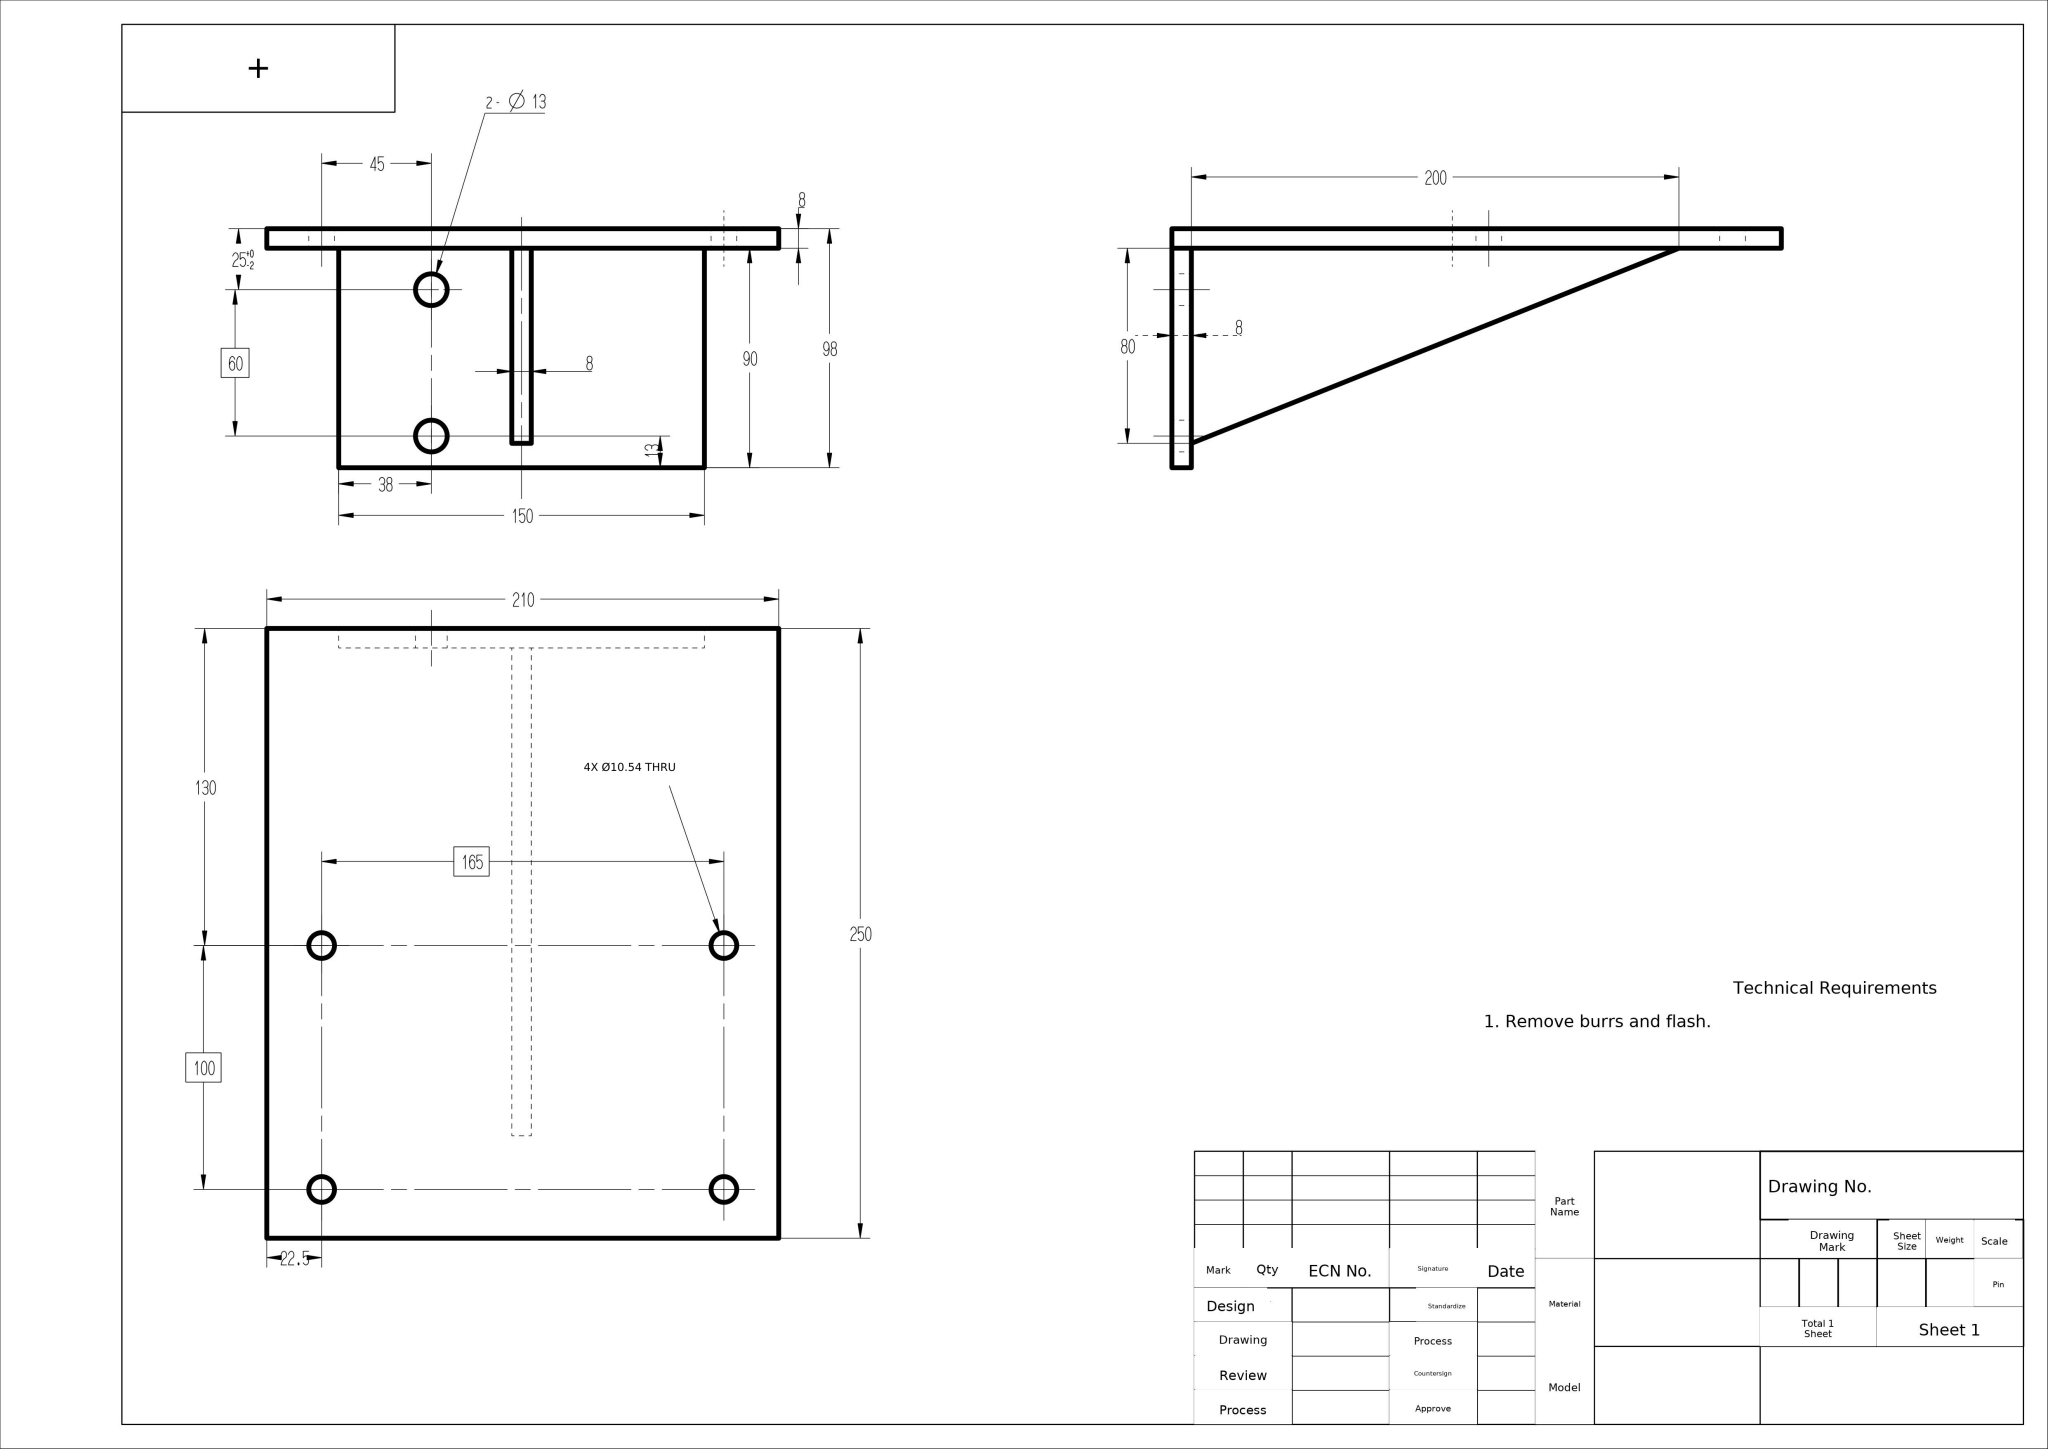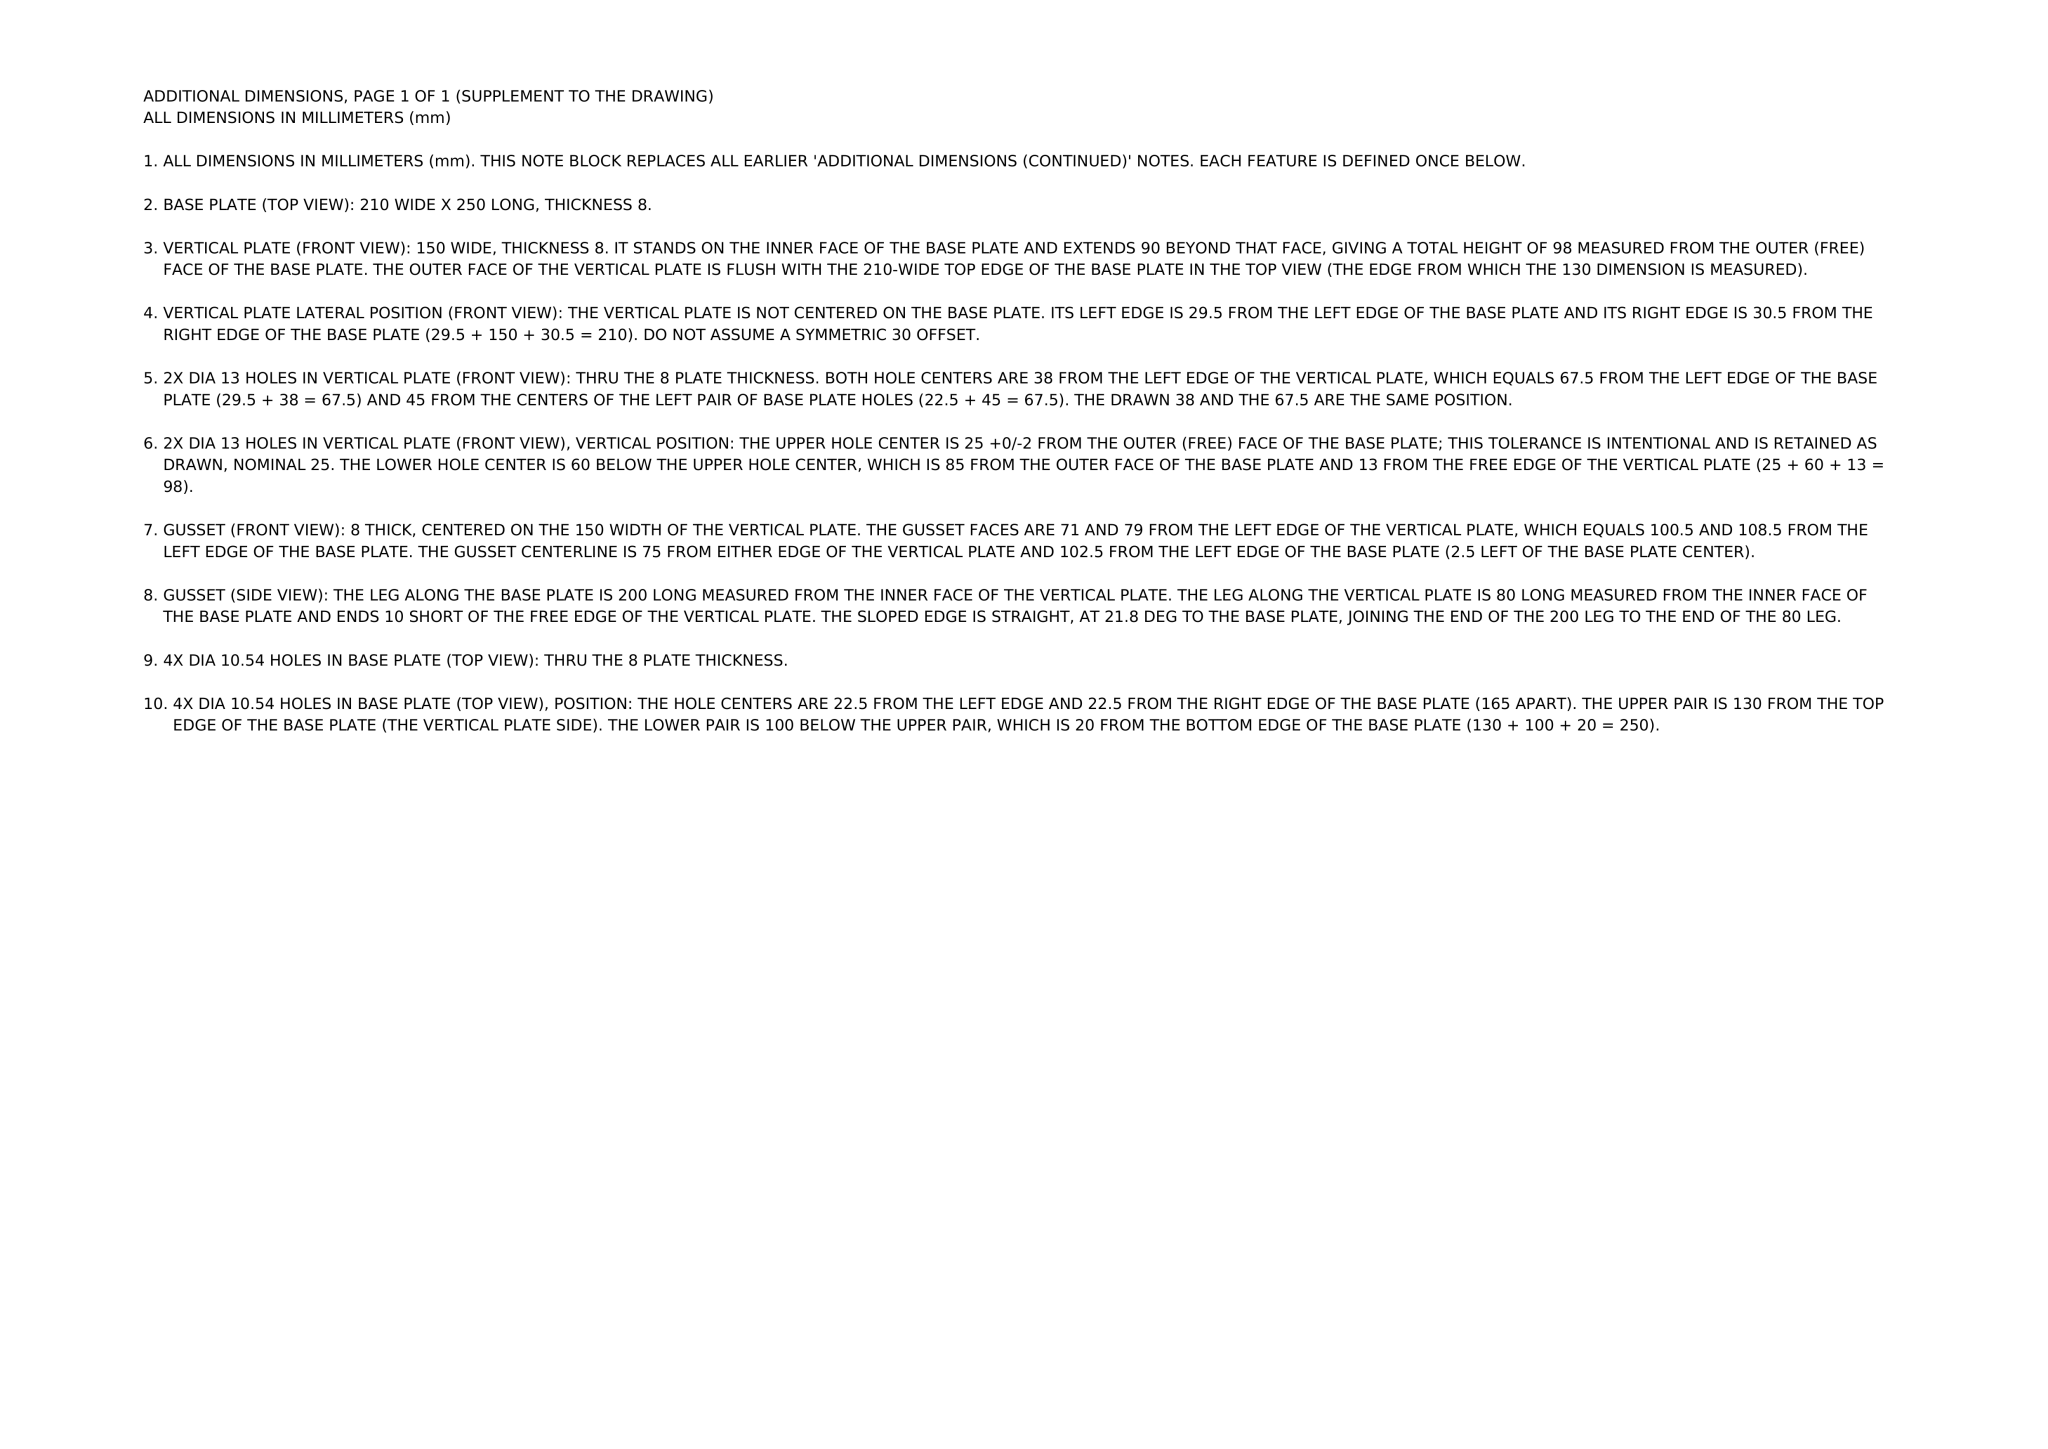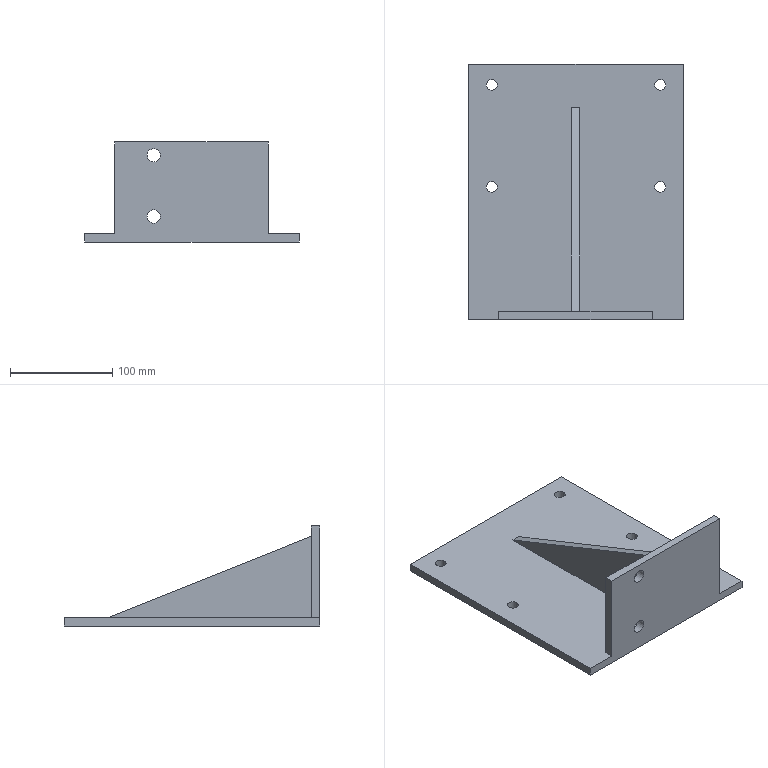Part | NX | mm | 1 solid | 19 faces | box 210 x 250 x 98 mm | volume 587086 mm3 | plane 13 | cylinder 6 | commonest cylinder face diameters 10.536 x4 13 x2
STEP:
#1=CARTESIAN_POINT('',(0.,0.,0.));
#2=DIRECTION('',(0.,0.,1.));
#3=DIRECTION('',(1.,0.,0.));
#4=AXIS2_PLACEMENT_3D('',#1,#2,#3);
#5=(LENGTH_UNIT()NAMED_UNIT(*)SI_UNIT(.MILLI.,.METRE.));
#6=UNCERTAINTY_MEASURE_WITH_UNIT(LENGTH_MEASURE(0.00002),#5,'','');
#7=(NAMED_UNIT(*)PLANE_ANGLE_UNIT()SI_UNIT($,.RADIAN.));
#8=PLANE_ANGLE_MEASURE_WITH_UNIT(PLANE_ANGLE_MEASURE(0.01745),#7);
#9=DIMENSIONAL_EXPONENTS(0.,0.,0.,0.,0.,0.,0.);
#10=(CONVERSION_BASED_UNIT('',#8)NAMED_UNIT(#9)PLANE_ANGLE_UNIT());
#11=(NAMED_UNIT(*)SI_UNIT($,.STERADIAN.)SOLID_ANGLE_UNIT());
#12=(GEOMETRIC_REPRESENTATION_CONTEXT(3)GLOBAL_UNCERTAINTY_ASSIGNED_CONTEXT((#6))GLOBAL_UNIT_ASSIGNED_CONTEXT((#5,#10,#11))REPRESENTATION_CONTEXT('',''));
#13=SHAPE_REPRESENTATION('',(#4),#12);
#14=CARTESIAN_POINT('',(72.,-239.1,85.));
#15=VERTEX_POINT('',#14);
#16=CARTESIAN_POINT('',(65.5,-239.1,85.));
#17=DIRECTION('',(0.,-1.,0.));
#18=DIRECTION('',(1.,0.,0.));
#19=AXIS2_PLACEMENT_3D('',#16,#17,#18);
#20=CIRCLE('',#19,6.5);
#21=EDGE_CURVE('',#15,#15,#20,.T.);
#22=ORIENTED_EDGE('',*,*,#21,.T.);
#23=EDGE_LOOP('',(#22));
#24=FACE_BOUND('',#23,.T.);
#25=CARTESIAN_POINT('',(72.,-239.1,25.));
#26=VERTEX_POINT('',#25);
#27=CARTESIAN_POINT('',(65.5,-239.1,25.));
#28=DIRECTION('',(0.,-1.,0.));
#29=DIRECTION('',(1.,0.,0.));
#30=AXIS2_PLACEMENT_3D('',#27,#28,#29);
#31=CIRCLE('',#30,6.5);
#32=EDGE_CURVE('',#26,#26,#31,.T.);
#33=ORIENTED_EDGE('',*,*,#32,.T.);
#34=EDGE_LOOP('',(#33));
#35=FACE_BOUND('',#34,.T.);
#36=CARTESIAN_POINT('',(177.5,-239.1,8.));
#37=VERTEX_POINT('',#36);
#38=CARTESIAN_POINT('',(106.5,-239.1,8.));
#39=VERTEX_POINT('',#38);
#40=CARTESIAN_POINT('',(177.5,-239.1,8.));
#41=DIRECTION('',(-1.,0.,0.));
#42=VECTOR('',#41,1.);
#43=LINE('',#40,#42);
#44=EDGE_CURVE('',#37,#39,#43,.T.);
#45=ORIENTED_EDGE('',*,*,#44,.T.);
#46=CARTESIAN_POINT('',(106.5,-239.1,88.));
#47=VERTEX_POINT('',#46);
#48=CARTESIAN_POINT('',(106.5,-239.1,8.));
#49=DIRECTION('',(0.,0.,1.));
#50=VECTOR('',#49,1.);
#51=LINE('',#48,#50);
#52=EDGE_CURVE('',#39,#47,#51,.T.);
#53=ORIENTED_EDGE('',*,*,#52,.T.);
#54=CARTESIAN_POINT('',(98.5,-239.1,88.));
#55=VERTEX_POINT('',#54);
#56=CARTESIAN_POINT('',(106.5,-239.1,88.));
#57=DIRECTION('',(-1.,0.,0.));
#58=VECTOR('',#57,1.);
#59=LINE('',#56,#58);
#60=EDGE_CURVE('',#47,#55,#59,.T.);
#61=ORIENTED_EDGE('',*,*,#60,.T.);
#62=CARTESIAN_POINT('',(98.5,-239.1,8.));
#63=VERTEX_POINT('',#62);
#64=CARTESIAN_POINT('',(98.5,-239.1,88.));
#65=DIRECTION('',(0.,0.,-1.));
#66=VECTOR('',#65,1.);
#67=LINE('',#64,#66);
#68=EDGE_CURVE('',#55,#63,#67,.T.);
#69=ORIENTED_EDGE('',*,*,#68,.T.);
#70=CARTESIAN_POINT('',(27.5,-239.1,8.));
#71=VERTEX_POINT('',#70);
#72=CARTESIAN_POINT('',(177.5,-239.1,8.));
#73=DIRECTION('',(-1.,0.,0.));
#74=VECTOR('',#73,1.);
#75=LINE('',#72,#74);
#76=EDGE_CURVE('',#63,#71,#75,.T.);
#77=ORIENTED_EDGE('',*,*,#76,.T.);
#78=CARTESIAN_POINT('',(27.5,-239.1,98.));
#79=VERTEX_POINT('',#78);
#80=CARTESIAN_POINT('',(27.5,-239.1,8.));
#81=DIRECTION('',(0.,0.,1.));
#82=VECTOR('',#81,1.);
#83=LINE('',#80,#82);
#84=EDGE_CURVE('',#71,#79,#83,.T.);
#85=ORIENTED_EDGE('',*,*,#84,.T.);
#86=CARTESIAN_POINT('',(177.5,-239.1,98.));
#87=VERTEX_POINT('',#86);
#88=CARTESIAN_POINT('',(27.5,-239.1,98.));
#89=DIRECTION('',(1.,0.,-0.));
#90=VECTOR('',#89,1.);
#91=LINE('',#88,#90);
#92=EDGE_CURVE('',#79,#87,#91,.T.);
#93=ORIENTED_EDGE('',*,*,#92,.T.);
#94=CARTESIAN_POINT('',(177.5,-239.1,98.));
#95=DIRECTION('',(-0.,0.,-1.));
#96=VECTOR('',#95,1.);
#97=LINE('',#94,#96);
#98=EDGE_CURVE('',#87,#37,#97,.T.);
#99=ORIENTED_EDGE('',*,*,#98,.T.);
#100=EDGE_LOOP('',(#45,#53,#61,#69,#77,#85,#93,#99));
#101=FACE_BOUND('',#100,.T.);
#102=CARTESIAN_POINT('',(65.5,-239.1,85.));
#103=DIRECTION('',(0.,-1.,0.));
#104=DIRECTION('',(0.,0.,-1.));
#105=AXIS2_PLACEMENT_3D('',#102,#103,#104);
#106=PLANE('',#105);
#107=ADVANCED_FACE('',(#24,#35,#101),#106,.F.);
#108=CARTESIAN_POINT('',(98.5,-39.1,8.));
#109=VERTEX_POINT('',#108);
#110=CARTESIAN_POINT('',(98.5,-39.1,8.));
#111=DIRECTION('',(0.,-1.,0.));
#112=VECTOR('',#111,1.);
#113=LINE('',#110,#112);
#114=EDGE_CURVE('',#109,#63,#113,.T.);
#115=ORIENTED_EDGE('',*,*,#114,.F.);
#116=CARTESIAN_POINT('',(106.5,-39.1,8.));
#117=VERTEX_POINT('',#116);
#118=CARTESIAN_POINT('',(98.5,-39.1,8.));
#119=DIRECTION('',(1.,0.,0.));
#120=VECTOR('',#119,1.);
#121=LINE('',#118,#120);
#122=EDGE_CURVE('',#109,#117,#121,.T.);
#123=ORIENTED_EDGE('',*,*,#122,.T.);
#124=CARTESIAN_POINT('',(106.5,-39.1,8.));
#125=DIRECTION('',(0.,-1.,0.));
#126=VECTOR('',#125,1.);
#127=LINE('',#124,#126);
#128=EDGE_CURVE('',#117,#39,#127,.T.);
#129=ORIENTED_EDGE('',*,*,#128,.T.);
#130=ORIENTED_EDGE('',*,*,#44,.F.);
#131=CARTESIAN_POINT('',(177.5,-247.1,8.));
#132=VERTEX_POINT('',#131);
#133=CARTESIAN_POINT('',(177.5,-239.1,8.));
#134=DIRECTION('',(0.,-1.,0.));
#135=VECTOR('',#134,1.);
#136=LINE('',#133,#135);
#137=EDGE_CURVE('',#37,#132,#136,.T.);
#138=ORIENTED_EDGE('',*,*,#137,.T.);
#139=CARTESIAN_POINT('',(208.,-247.1,8.));
#140=VERTEX_POINT('',#139);
#141=CARTESIAN_POINT('',(208.,-247.1,8.));
#142=DIRECTION('',(-1.,0.,0.));
#143=VECTOR('',#142,1.);
#144=LINE('',#141,#143);
#145=EDGE_CURVE('',#140,#132,#144,.T.);
#146=ORIENTED_EDGE('',*,*,#145,.F.);
#147=CARTESIAN_POINT('',(208.,2.9,8.));
#148=VERTEX_POINT('',#147);
#149=CARTESIAN_POINT('',(208.,2.9,8.));
#150=DIRECTION('',(0.,-1.,0.));
#151=VECTOR('',#150,1.);
#152=LINE('',#149,#151);
#153=EDGE_CURVE('',#148,#140,#152,.T.);
#154=ORIENTED_EDGE('',*,*,#153,.F.);
#155=CARTESIAN_POINT('',(-2.,2.9,8.));
#156=VERTEX_POINT('',#155);
#157=CARTESIAN_POINT('',(-2.,2.9,8.));
#158=DIRECTION('',(1.,-0.,0.));
#159=VECTOR('',#158,1.);
#160=LINE('',#157,#159);
#161=EDGE_CURVE('',#156,#148,#160,.T.);
#162=ORIENTED_EDGE('',*,*,#161,.F.);
#163=CARTESIAN_POINT('',(-2.,-247.1,8.));
#164=VERTEX_POINT('',#163);
#165=CARTESIAN_POINT('',(-2.,-247.1,8.));
#166=DIRECTION('',(-0.,1.,0.));
#167=VECTOR('',#166,1.);
#168=LINE('',#165,#167);
#169=EDGE_CURVE('',#164,#156,#168,.T.);
#170=ORIENTED_EDGE('',*,*,#169,.F.);
#171=CARTESIAN_POINT('',(27.5,-247.1,8.));
#172=VERTEX_POINT('',#171);
#173=CARTESIAN_POINT('',(208.,-247.1,8.));
#174=DIRECTION('',(-1.,0.,0.));
#175=VECTOR('',#174,1.);
#176=LINE('',#173,#175);
#177=EDGE_CURVE('',#172,#164,#176,.T.);
#178=ORIENTED_EDGE('',*,*,#177,.F.);
#179=CARTESIAN_POINT('',(27.5,-239.1,8.));
#180=DIRECTION('',(0.,-1.,0.));
#181=VECTOR('',#180,1.);
#182=LINE('',#179,#181);
#183=EDGE_CURVE('',#71,#172,#182,.T.);
#184=ORIENTED_EDGE('',*,*,#183,.F.);
#185=ORIENTED_EDGE('',*,*,#76,.F.);
#186=EDGE_LOOP('',(#115,#123,#129,#130,#138,#146,#154,#162,#170,#178,#184,#185));
#187=FACE_BOUND('',#186,.T.);
#188=CARTESIAN_POINT('',(190.768,-17.1,8.));
#189=VERTEX_POINT('',#188);
#190=CARTESIAN_POINT('',(185.5,-17.1,8.));
#191=DIRECTION('',(0.,0.,1.));
#192=DIRECTION('',(1.,0.,0.));
#193=AXIS2_PLACEMENT_3D('',#190,#191,#192);
#194=CIRCLE('',#193,5.268);
#195=EDGE_CURVE('',#189,#189,#194,.T.);
#196=ORIENTED_EDGE('',*,*,#195,.F.);
#197=EDGE_LOOP('',(#196));
#198=FACE_BOUND('',#197,.T.);
#199=CARTESIAN_POINT('',(190.768,-117.1,8.));
#200=VERTEX_POINT('',#199);
#201=CARTESIAN_POINT('',(185.5,-117.1,8.));
#202=DIRECTION('',(0.,0.,1.));
#203=DIRECTION('',(1.,0.,0.));
#204=AXIS2_PLACEMENT_3D('',#201,#202,#203);
#205=CIRCLE('',#204,5.268);
#206=EDGE_CURVE('',#200,#200,#205,.T.);
#207=ORIENTED_EDGE('',*,*,#206,.F.);
#208=EDGE_LOOP('',(#207));
#209=FACE_BOUND('',#208,.T.);
#210=CARTESIAN_POINT('',(25.768,-17.1,8.));
#211=VERTEX_POINT('',#210);
#212=CARTESIAN_POINT('',(20.5,-17.1,8.));
#213=DIRECTION('',(0.,0.,1.));
#214=DIRECTION('',(1.,0.,0.));
#215=AXIS2_PLACEMENT_3D('',#212,#213,#214);
#216=CIRCLE('',#215,5.268);
#217=EDGE_CURVE('',#211,#211,#216,.T.);
#218=ORIENTED_EDGE('',*,*,#217,.F.);
#219=EDGE_LOOP('',(#218));
#220=FACE_BOUND('',#219,.T.);
#221=CARTESIAN_POINT('',(25.768,-117.1,8.));
#222=VERTEX_POINT('',#221);
#223=CARTESIAN_POINT('',(20.5,-117.1,8.));
#224=DIRECTION('',(0.,0.,-1.));
#225=DIRECTION('',(1.,0.,0.));
#226=AXIS2_PLACEMENT_3D('',#223,#224,#225);
#227=CIRCLE('',#226,5.268);
#228=EDGE_CURVE('',#222,#222,#227,.T.);
#229=ORIENTED_EDGE('',*,*,#228,.T.);
#230=EDGE_LOOP('',(#229));
#231=FACE_BOUND('',#230,.T.);
#232=CARTESIAN_POINT('',(0.,0.,8.));
#233=DIRECTION('',(0.,0.,-1.));
#234=DIRECTION('',(-1.,0.,0.));
#235=AXIS2_PLACEMENT_3D('',#232,#233,#234);
#236=PLANE('',#235);
#237=ADVANCED_FACE('',(#187,#198,#209,#220,#231),#236,.F.);
#238=CARTESIAN_POINT('',(-2.,2.9,0.));
#239=VERTEX_POINT('',#238);
#240=CARTESIAN_POINT('',(208.,2.9,0.));
#241=VERTEX_POINT('',#240);
#242=CARTESIAN_POINT('',(-2.,2.9,0.));
#243=DIRECTION('',(1.,-0.,0.));
#244=VECTOR('',#243,1.);
#245=LINE('',#242,#244);
#246=EDGE_CURVE('',#239,#241,#245,.T.);
#247=ORIENTED_EDGE('',*,*,#246,.F.);
#248=CARTESIAN_POINT('',(-2.,2.9,8.));
#249=DIRECTION('',(0.,0.,-1.));
#250=VECTOR('',#249,1.);
#251=LINE('',#248,#250);
#252=EDGE_CURVE('',#156,#239,#251,.T.);
#253=ORIENTED_EDGE('',*,*,#252,.F.);
#254=ORIENTED_EDGE('',*,*,#161,.T.);
#255=CARTESIAN_POINT('',(208.,2.9,8.));
#256=DIRECTION('',(0.,0.,-1.));
#257=VECTOR('',#256,1.);
#258=LINE('',#255,#257);
#259=EDGE_CURVE('',#148,#241,#258,.T.);
#260=ORIENTED_EDGE('',*,*,#259,.T.);
#261=EDGE_LOOP('',(#247,#253,#254,#260));
#262=FACE_OUTER_BOUND('',#261,.T.);
#263=CARTESIAN_POINT('',(-2.,2.9,8.));
#264=DIRECTION('',(0.,1.,0.));
#265=DIRECTION('',(-1.,0.,0.));
#266=AXIS2_PLACEMENT_3D('',#263,#264,#265);
#267=PLANE('',#266);
#268=ADVANCED_FACE('',(#262),#267,.T.);
#269=CARTESIAN_POINT('',(208.,-247.1,0.));
#270=VERTEX_POINT('',#269);
#271=CARTESIAN_POINT('',(208.,2.9,0.));
#272=DIRECTION('',(0.,-1.,0.));
#273=VECTOR('',#272,1.);
#274=LINE('',#271,#273);
#275=EDGE_CURVE('',#241,#270,#274,.T.);
#276=ORIENTED_EDGE('',*,*,#275,.F.);
#277=ORIENTED_EDGE('',*,*,#259,.F.);
#278=ORIENTED_EDGE('',*,*,#153,.T.);
#279=CARTESIAN_POINT('',(208.,-247.1,8.));
#280=DIRECTION('',(0.,0.,-1.));
#281=VECTOR('',#280,1.);
#282=LINE('',#279,#281);
#283=EDGE_CURVE('',#140,#270,#282,.T.);
#284=ORIENTED_EDGE('',*,*,#283,.T.);
#285=EDGE_LOOP('',(#276,#277,#278,#284));
#286=FACE_OUTER_BOUND('',#285,.T.);
#287=CARTESIAN_POINT('',(208.,2.9,8.));
#288=DIRECTION('',(1.,0.,0.));
#289=DIRECTION('',(-0.,1.,0.));
#290=AXIS2_PLACEMENT_3D('',#287,#288,#289);
#291=PLANE('',#290);
#292=ADVANCED_FACE('',(#286),#291,.T.);
#293=CARTESIAN_POINT('',(-2.,-247.1,0.));
#294=VERTEX_POINT('',#293);
#295=CARTESIAN_POINT('',(208.,-247.1,0.));
#296=DIRECTION('',(-1.,0.,0.));
#297=VECTOR('',#296,1.);
#298=LINE('',#295,#297);
#299=EDGE_CURVE('',#270,#294,#298,.T.);
#300=ORIENTED_EDGE('',*,*,#299,.F.);
#301=ORIENTED_EDGE('',*,*,#283,.F.);
#302=ORIENTED_EDGE('',*,*,#145,.T.);
#303=CARTESIAN_POINT('',(177.5,-247.1,98.));
#304=VERTEX_POINT('',#303);
#305=CARTESIAN_POINT('',(177.5,-247.1,98.));
#306=DIRECTION('',(-0.,0.,-1.));
#307=VECTOR('',#306,1.);
#308=LINE('',#305,#307);
#309=EDGE_CURVE('',#304,#132,#308,.T.);
#310=ORIENTED_EDGE('',*,*,#309,.F.);
#311=CARTESIAN_POINT('',(27.5,-247.1,98.));
#312=VERTEX_POINT('',#311);
#313=CARTESIAN_POINT('',(27.5,-247.1,98.));
#314=DIRECTION('',(1.,0.,-0.));
#315=VECTOR('',#314,1.);
#316=LINE('',#313,#315);
#317=EDGE_CURVE('',#312,#304,#316,.T.);
#318=ORIENTED_EDGE('',*,*,#317,.F.);
#319=CARTESIAN_POINT('',(27.5,-247.1,8.));
#320=DIRECTION('',(0.,0.,1.));
#321=VECTOR('',#320,1.);
#322=LINE('',#319,#321);
#323=EDGE_CURVE('',#172,#312,#322,.T.);
#324=ORIENTED_EDGE('',*,*,#323,.F.);
#325=ORIENTED_EDGE('',*,*,#177,.T.);
#326=CARTESIAN_POINT('',(-2.,-247.1,8.));
#327=DIRECTION('',(0.,0.,-1.));
#328=VECTOR('',#327,1.);
#329=LINE('',#326,#328);
#330=EDGE_CURVE('',#164,#294,#329,.T.);
#331=ORIENTED_EDGE('',*,*,#330,.T.);
#332=EDGE_LOOP('',(#300,#301,#302,#310,#318,#324,#325,#331));
#333=FACE_BOUND('',#332,.T.);
#334=CARTESIAN_POINT('',(72.,-247.1,85.));
#335=VERTEX_POINT('',#334);
#336=CARTESIAN_POINT('',(65.5,-247.1,85.));
#337=DIRECTION('',(0.,-1.,0.));
#338=DIRECTION('',(1.,0.,0.));
#339=AXIS2_PLACEMENT_3D('',#336,#337,#338);
#340=CIRCLE('',#339,6.5);
#341=EDGE_CURVE('',#335,#335,#340,.T.);
#342=ORIENTED_EDGE('',*,*,#341,.F.);
#343=EDGE_LOOP('',(#342));
#344=FACE_BOUND('',#343,.T.);
#345=CARTESIAN_POINT('',(72.,-247.1,25.));
#346=VERTEX_POINT('',#345);
#347=CARTESIAN_POINT('',(65.5,-247.1,25.));
#348=DIRECTION('',(0.,-1.,0.));
#349=DIRECTION('',(1.,0.,0.));
#350=AXIS2_PLACEMENT_3D('',#347,#348,#349);
#351=CIRCLE('',#350,6.5);
#352=EDGE_CURVE('',#346,#346,#351,.T.);
#353=ORIENTED_EDGE('',*,*,#352,.F.);
#354=EDGE_LOOP('',(#353));
#355=FACE_BOUND('',#354,.T.);
#356=CARTESIAN_POINT('',(208.,-247.1,8.));
#357=DIRECTION('',(0.,-1.,0.));
#358=DIRECTION('',(0.,0.,-1.));
#359=AXIS2_PLACEMENT_3D('',#356,#357,#358);
#360=PLANE('',#359);
#361=ADVANCED_FACE('',(#333,#344,#355),#360,.T.);
#362=CARTESIAN_POINT('',(-2.,-247.1,0.));
#363=DIRECTION('',(-0.,1.,0.));
#364=VECTOR('',#363,1.);
#365=LINE('',#362,#364);
#366=EDGE_CURVE('',#294,#239,#365,.T.);
#367=ORIENTED_EDGE('',*,*,#366,.F.);
#368=ORIENTED_EDGE('',*,*,#330,.F.);
#369=ORIENTED_EDGE('',*,*,#169,.T.);
#370=ORIENTED_EDGE('',*,*,#252,.T.);
#371=EDGE_LOOP('',(#367,#368,#369,#370));
#372=FACE_OUTER_BOUND('',#371,.T.);
#373=CARTESIAN_POINT('',(-2.,-247.1,8.));
#374=DIRECTION('',(-1.,-0.,0.));
#375=DIRECTION('',(0.,-1.,0.));
#376=AXIS2_PLACEMENT_3D('',#373,#374,#375);
#377=PLANE('',#376);
#378=ADVANCED_FACE('',(#372),#377,.T.);
#379=CARTESIAN_POINT('',(25.768,-117.1,0.));
#380=VERTEX_POINT('',#379);
#381=CARTESIAN_POINT('',(20.5,-117.1,0.));
#382=DIRECTION('',(0.,0.,-1.));
#383=DIRECTION('',(1.,0.,0.));
#384=AXIS2_PLACEMENT_3D('',#381,#382,#383);
#385=CIRCLE('',#384,5.268);
#386=EDGE_CURVE('',#380,#380,#385,.T.);
#387=ORIENTED_EDGE('',*,*,#386,.F.);
#388=EDGE_LOOP('',(#387));
#389=FACE_BOUND('',#388,.T.);
#390=CARTESIAN_POINT('',(25.768,-17.1,0.));
#391=VERTEX_POINT('',#390);
#392=CARTESIAN_POINT('',(20.5,-17.1,0.));
#393=DIRECTION('',(0.,0.,1.));
#394=DIRECTION('',(1.,0.,0.));
#395=AXIS2_PLACEMENT_3D('',#392,#393,#394);
#396=CIRCLE('',#395,5.268);
#397=EDGE_CURVE('',#391,#391,#396,.T.);
#398=ORIENTED_EDGE('',*,*,#397,.T.);
#399=EDGE_LOOP('',(#398));
#400=FACE_BOUND('',#399,.T.);
#401=CARTESIAN_POINT('',(190.768,-117.1,0.));
#402=VERTEX_POINT('',#401);
#403=CARTESIAN_POINT('',(185.5,-117.1,0.));
#404=DIRECTION('',(0.,0.,1.));
#405=DIRECTION('',(1.,0.,0.));
#406=AXIS2_PLACEMENT_3D('',#403,#404,#405);
#407=CIRCLE('',#406,5.268);
#408=EDGE_CURVE('',#402,#402,#407,.T.);
#409=ORIENTED_EDGE('',*,*,#408,.T.);
#410=EDGE_LOOP('',(#409));
#411=FACE_BOUND('',#410,.T.);
#412=CARTESIAN_POINT('',(190.768,-17.1,0.));
#413=VERTEX_POINT('',#412);
#414=CARTESIAN_POINT('',(185.5,-17.1,0.));
#415=DIRECTION('',(0.,0.,1.));
#416=DIRECTION('',(1.,0.,0.));
#417=AXIS2_PLACEMENT_3D('',#414,#415,#416);
#418=CIRCLE('',#417,5.268);
#419=EDGE_CURVE('',#413,#413,#418,.T.);
#420=ORIENTED_EDGE('',*,*,#419,.T.);
#421=EDGE_LOOP('',(#420));
#422=FACE_BOUND('',#421,.T.);
#423=ORIENTED_EDGE('',*,*,#246,.T.);
#424=ORIENTED_EDGE('',*,*,#275,.T.);
#425=ORIENTED_EDGE('',*,*,#299,.T.);
#426=ORIENTED_EDGE('',*,*,#366,.T.);
#427=EDGE_LOOP('',(#423,#424,#425,#426));
#428=FACE_BOUND('',#427,.T.);
#429=CARTESIAN_POINT('',(0.,0.,0.));
#430=DIRECTION('',(0.,0.,-1.));
#431=DIRECTION('',(-1.,0.,0.));
#432=AXIS2_PLACEMENT_3D('',#429,#430,#431);
#433=PLANE('',#432);
#434=ADVANCED_FACE('',(#389,#400,#411,#422,#428),#433,.T.);
#435=ORIENTED_EDGE('',*,*,#195,.T.);
#436=EDGE_LOOP('',(#435));
#437=FACE_BOUND('',#436,.T.);
#438=ORIENTED_EDGE('',*,*,#419,.F.);
#439=EDGE_LOOP('',(#438));
#440=FACE_BOUND('',#439,.T.);
#441=CARTESIAN_POINT('',(185.5,-17.1,8.));
#442=DIRECTION('',(0.,0.,-1.));
#443=DIRECTION('',(-1.,0.,0.));
#444=AXIS2_PLACEMENT_3D('',#441,#442,#443);
#445=CYLINDRICAL_SURFACE('',#444,5.268);
#446=ADVANCED_FACE('',(#437,#440),#445,.F.);
#447=ORIENTED_EDGE('',*,*,#206,.T.);
#448=EDGE_LOOP('',(#447));
#449=FACE_BOUND('',#448,.T.);
#450=ORIENTED_EDGE('',*,*,#408,.F.);
#451=EDGE_LOOP('',(#450));
#452=FACE_BOUND('',#451,.T.);
#453=CARTESIAN_POINT('',(185.5,-117.1,8.));
#454=DIRECTION('',(0.,0.,-1.));
#455=DIRECTION('',(-1.,0.,0.));
#456=AXIS2_PLACEMENT_3D('',#453,#454,#455);
#457=CYLINDRICAL_SURFACE('',#456,5.268);
#458=ADVANCED_FACE('',(#449,#452),#457,.F.);
#459=ORIENTED_EDGE('',*,*,#217,.T.);
#460=EDGE_LOOP('',(#459));
#461=FACE_BOUND('',#460,.T.);
#462=ORIENTED_EDGE('',*,*,#397,.F.);
#463=EDGE_LOOP('',(#462));
#464=FACE_BOUND('',#463,.T.);
#465=CARTESIAN_POINT('',(20.5,-17.1,8.));
#466=DIRECTION('',(0.,0.,-1.));
#467=DIRECTION('',(-1.,0.,0.));
#468=AXIS2_PLACEMENT_3D('',#465,#466,#467);
#469=CYLINDRICAL_SURFACE('',#468,5.268);
#470=ADVANCED_FACE('',(#461,#464),#469,.F.);
#471=ORIENTED_EDGE('',*,*,#228,.F.);
#472=EDGE_LOOP('',(#471));
#473=FACE_BOUND('',#472,.T.);
#474=ORIENTED_EDGE('',*,*,#386,.T.);
#475=EDGE_LOOP('',(#474));
#476=FACE_BOUND('',#475,.T.);
#477=CARTESIAN_POINT('',(20.5,-117.1,8.));
#478=DIRECTION('',(0.,0.,-1.));
#479=DIRECTION('',(-1.,0.,0.));
#480=AXIS2_PLACEMENT_3D('',#477,#478,#479);
#481=CYLINDRICAL_SURFACE('',#480,5.268);
#482=ADVANCED_FACE('',(#473,#476),#481,.F.);
#483=ORIENTED_EDGE('',*,*,#323,.T.);
#484=CARTESIAN_POINT('',(27.5,-239.1,98.));
#485=DIRECTION('',(0.,-1.,0.));
#486=VECTOR('',#485,1.);
#487=LINE('',#484,#486);
#488=EDGE_CURVE('',#79,#312,#487,.T.);
#489=ORIENTED_EDGE('',*,*,#488,.F.);
#490=ORIENTED_EDGE('',*,*,#84,.F.);
#491=ORIENTED_EDGE('',*,*,#183,.T.);
#492=EDGE_LOOP('',(#483,#489,#490,#491));
#493=FACE_OUTER_BOUND('',#492,.T.);
#494=CARTESIAN_POINT('',(27.5,-239.1,8.));
#495=DIRECTION('',(1.,0.,0.));
#496=DIRECTION('',(0.,0.,-1.));
#497=AXIS2_PLACEMENT_3D('',#494,#495,#496);
#498=PLANE('',#497);
#499=ADVANCED_FACE('',(#493),#498,.F.);
#500=ORIENTED_EDGE('',*,*,#317,.T.);
#501=CARTESIAN_POINT('',(177.5,-239.1,98.));
#502=DIRECTION('',(0.,-1.,0.));
#503=VECTOR('',#502,1.);
#504=LINE('',#501,#503);
#505=EDGE_CURVE('',#87,#304,#504,.T.);
#506=ORIENTED_EDGE('',*,*,#505,.F.);
#507=ORIENTED_EDGE('',*,*,#92,.F.);
#508=ORIENTED_EDGE('',*,*,#488,.T.);
#509=EDGE_LOOP('',(#500,#506,#507,#508));
#510=FACE_OUTER_BOUND('',#509,.T.);
#511=CARTESIAN_POINT('',(27.5,-239.1,98.));
#512=DIRECTION('',(-0.,0.,-1.));
#513=DIRECTION('',(-1.,0.,0.));
#514=AXIS2_PLACEMENT_3D('',#511,#512,#513);
#515=PLANE('',#514);
#516=ADVANCED_FACE('',(#510),#515,.F.);
#517=ORIENTED_EDGE('',*,*,#309,.T.);
#518=ORIENTED_EDGE('',*,*,#137,.F.);
#519=ORIENTED_EDGE('',*,*,#98,.F.);
#520=ORIENTED_EDGE('',*,*,#505,.T.);
#521=EDGE_LOOP('',(#517,#518,#519,#520));
#522=FACE_OUTER_BOUND('',#521,.T.);
#523=CARTESIAN_POINT('',(177.5,-239.1,98.));
#524=DIRECTION('',(-1.,0.,0.));
#525=DIRECTION('',(0.,0.,1.));
#526=AXIS2_PLACEMENT_3D('',#523,#524,#525);
#527=PLANE('',#526);
#528=ADVANCED_FACE('',(#522),#527,.F.);
#529=ORIENTED_EDGE('',*,*,#21,.F.);
#530=EDGE_LOOP('',(#529));
#531=FACE_BOUND('',#530,.T.);
#532=ORIENTED_EDGE('',*,*,#341,.T.);
#533=EDGE_LOOP('',(#532));
#534=FACE_BOUND('',#533,.T.);
#535=CARTESIAN_POINT('',(65.5,-239.1,85.));
#536=DIRECTION('',(0.,-1.,0.));
#537=DIRECTION('',(0.,0.,-1.));
#538=AXIS2_PLACEMENT_3D('',#535,#536,#537);
#539=CYLINDRICAL_SURFACE('',#538,6.5);
#540=ADVANCED_FACE('',(#531,#534),#539,.F.);
#541=ORIENTED_EDGE('',*,*,#32,.F.);
#542=EDGE_LOOP('',(#541));
#543=FACE_BOUND('',#542,.T.);
#544=ORIENTED_EDGE('',*,*,#352,.T.);
#545=EDGE_LOOP('',(#544));
#546=FACE_BOUND('',#545,.T.);
#547=CARTESIAN_POINT('',(65.5,-239.1,25.));
#548=DIRECTION('',(0.,-1.,0.));
#549=DIRECTION('',(0.,0.,-1.));
#550=AXIS2_PLACEMENT_3D('',#547,#548,#549);
#551=CYLINDRICAL_SURFACE('',#550,6.5);
#552=ADVANCED_FACE('',(#543,#546),#551,.F.);
#553=CARTESIAN_POINT('',(106.5,-39.1,8.));
#554=DIRECTION('',(-0.,0.9285,-0.3714));
#555=VECTOR('',#554,1.);
#556=LINE('',#553,#555);
#557=EDGE_CURVE('',#47,#117,#556,.T.);
#558=ORIENTED_EDGE('',*,*,#557,.F.);
#559=ORIENTED_EDGE('',*,*,#52,.F.);
#560=ORIENTED_EDGE('',*,*,#128,.F.);
#561=EDGE_LOOP('',(#558,#559,#560));
#562=FACE_OUTER_BOUND('',#561,.T.);
#563=CARTESIAN_POINT('',(106.5,-39.1,8.));
#564=DIRECTION('',(1.,0.,-0.));
#565=DIRECTION('',(-0.,0.,-1.));
#566=AXIS2_PLACEMENT_3D('',#563,#564,#565);
#567=PLANE('',#566);
#568=ADVANCED_FACE('',(#562),#567,.T.);
#569=CARTESIAN_POINT('',(98.5,-66.686,19.034));
#570=DIRECTION('',(0.,-0.9285,0.3714));
#571=VECTOR('',#570,1.);
#572=LINE('',#569,#571);
#573=EDGE_CURVE('',#109,#55,#572,.T.);
#574=ORIENTED_EDGE('',*,*,#573,.F.);
#575=ORIENTED_EDGE('',*,*,#114,.T.);
#576=ORIENTED_EDGE('',*,*,#68,.F.);
#577=EDGE_LOOP('',(#574,#575,#576));
#578=FACE_OUTER_BOUND('',#577,.T.);
#579=CARTESIAN_POINT('',(98.5,-39.1,88.));
#580=DIRECTION('',(-1.,0.,0.));
#581=DIRECTION('',(0.,0.,1.));
#582=AXIS2_PLACEMENT_3D('',#579,#580,#581);
#583=PLANE('',#582);
#584=ADVANCED_FACE('',(#578),#583,.T.);
#585=ORIENTED_EDGE('',*,*,#557,.T.);
#586=ORIENTED_EDGE('',*,*,#122,.F.);
#587=ORIENTED_EDGE('',*,*,#573,.T.);
#588=ORIENTED_EDGE('',*,*,#60,.F.);
#589=EDGE_LOOP('',(#585,#586,#587,#588));
#590=FACE_OUTER_BOUND('',#589,.T.);
#591=CARTESIAN_POINT('',(99.5,-114.1,38.));
#592=DIRECTION('',(-0.,-0.3714,-0.9285));
#593=DIRECTION('',(0.,0.9285,-0.3714));
#594=AXIS2_PLACEMENT_3D('',#591,#592,#593);
#595=PLANE('',#594);
#596=ADVANCED_FACE('',(#590),#595,.F.);
#597=CLOSED_SHELL('',(#107,#237,#268,#292,#361,#378,#434,#446,#458,#470,#482,#499,#516,#528,#540,#552,#568,#584,#596));
#598=MANIFOLD_SOLID_BREP('',#597);
#599=ADVANCED_BREP_SHAPE_REPRESENTATION('',(#598),#12);
#600=SHAPE_REPRESENTATION_RELATIONSHIP('','',#13,#599);
#601=PRESENTATION_LAYER_ASSIGNMENT('','',(#598));
#602=COLOUR_RGB('',1.,0.6,0.);
#603=FILL_AREA_STYLE_COLOUR('',#602);
#604=FILL_AREA_STYLE('',(#603));
#605=SURFACE_STYLE_FILL_AREA(#604);
#606=SURFACE_SIDE_STYLE('',(#605));
#607=SURFACE_STYLE_USAGE(.BOTH.,#606);
#608=PRESENTATION_STYLE_ASSIGNMENT((#607));
#609=STYLED_ITEM('',(#608),#598);
#610=MECHANICAL_DESIGN_GEOMETRIC_PRESENTATION_REPRESENTATION('',(#609),#12);